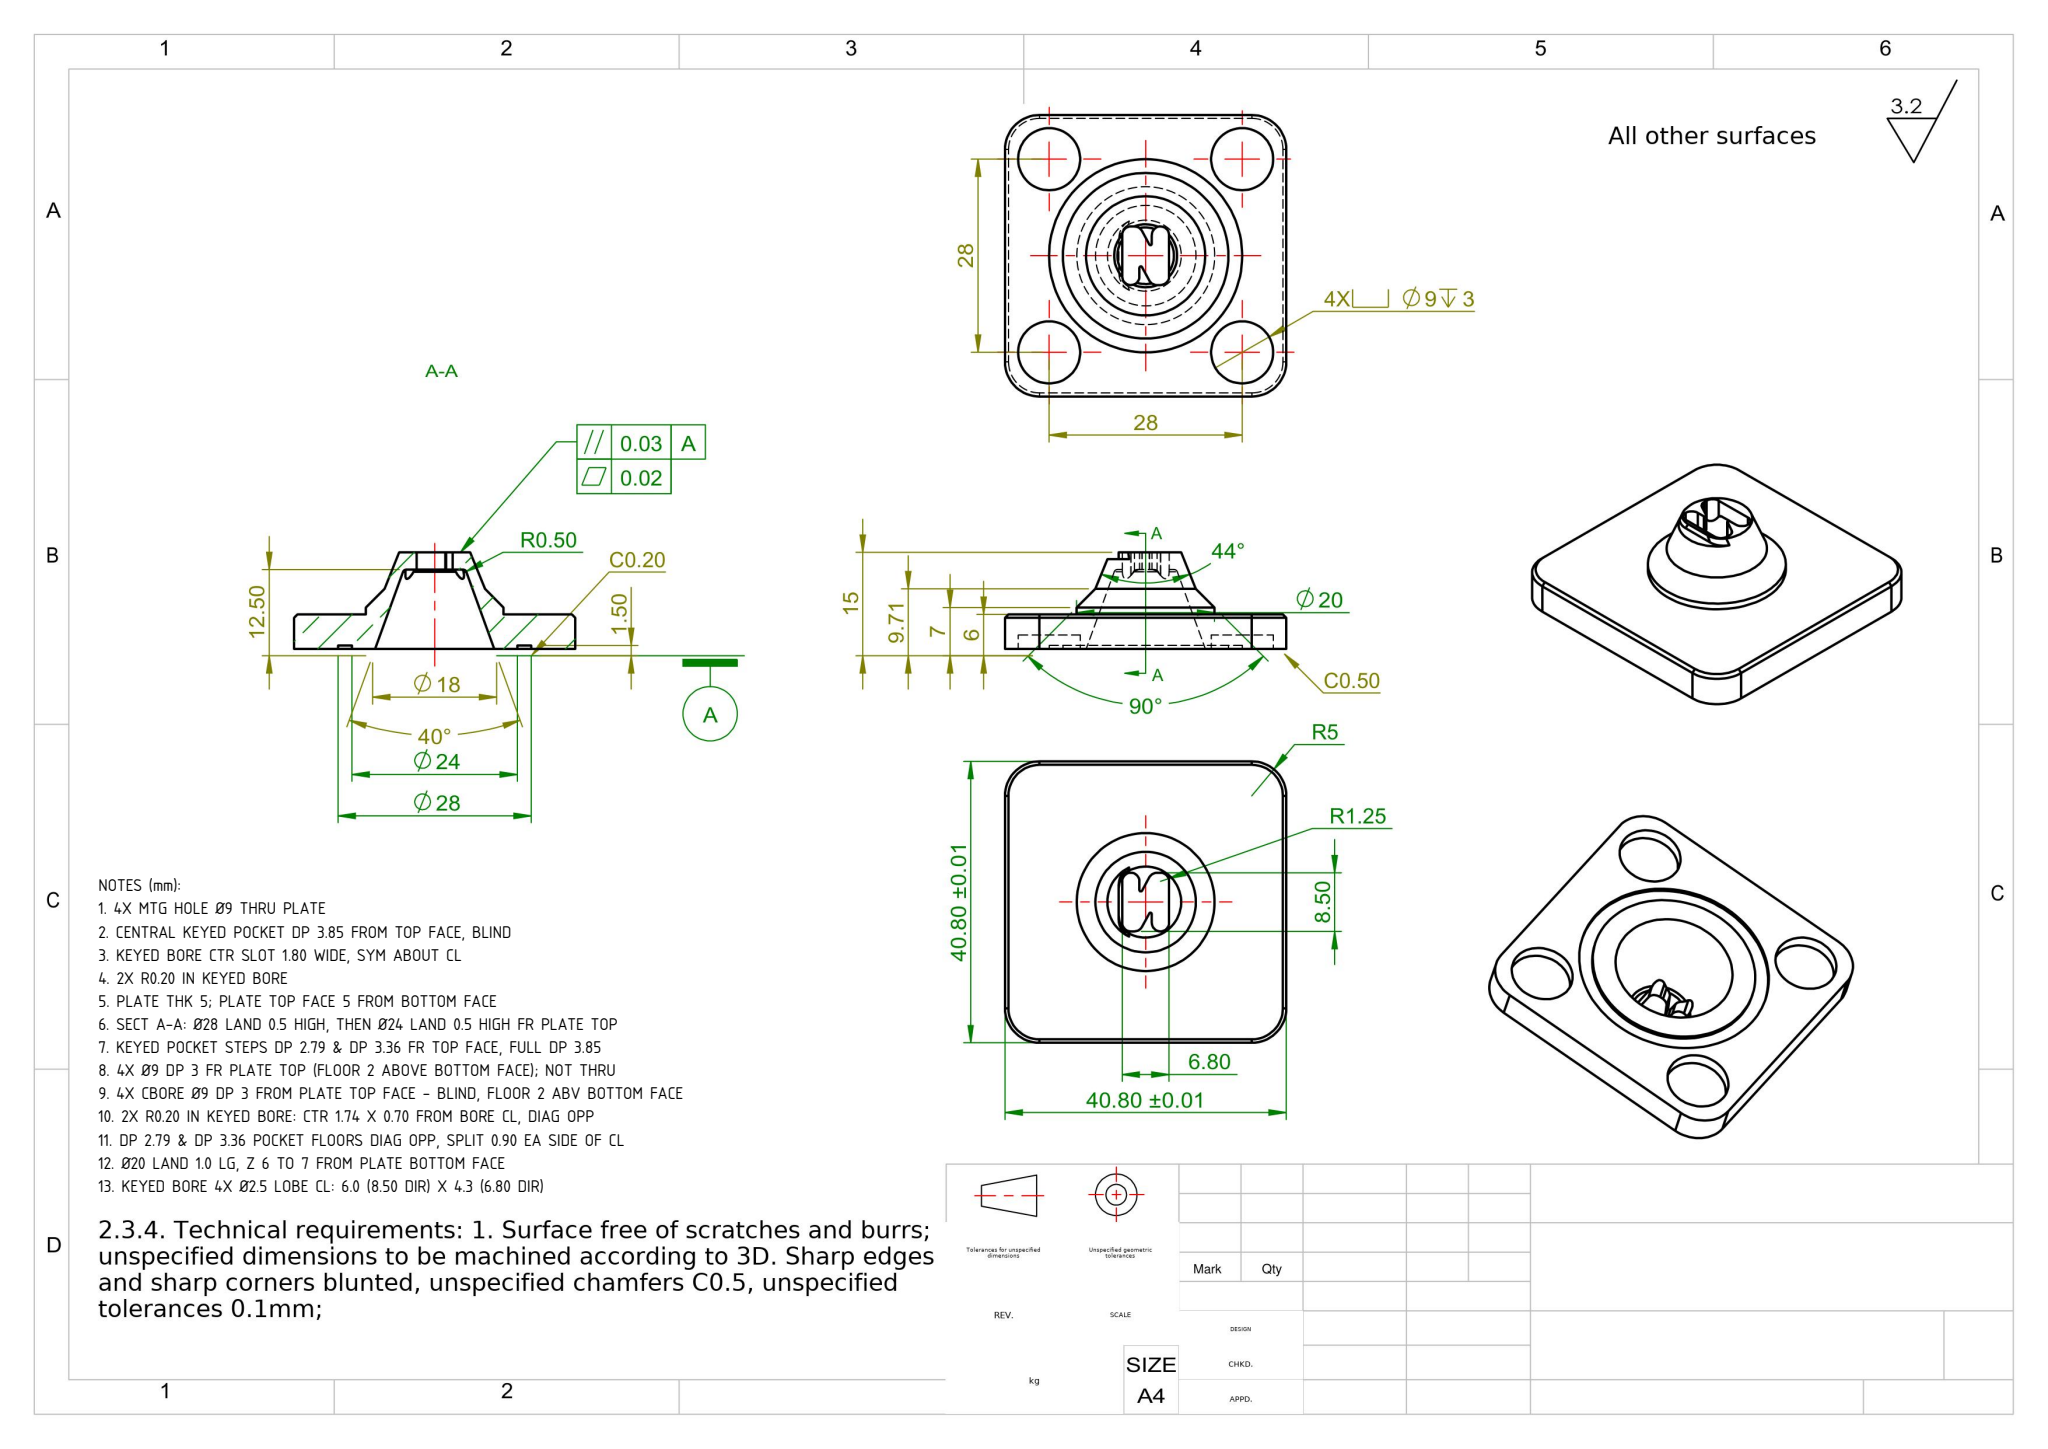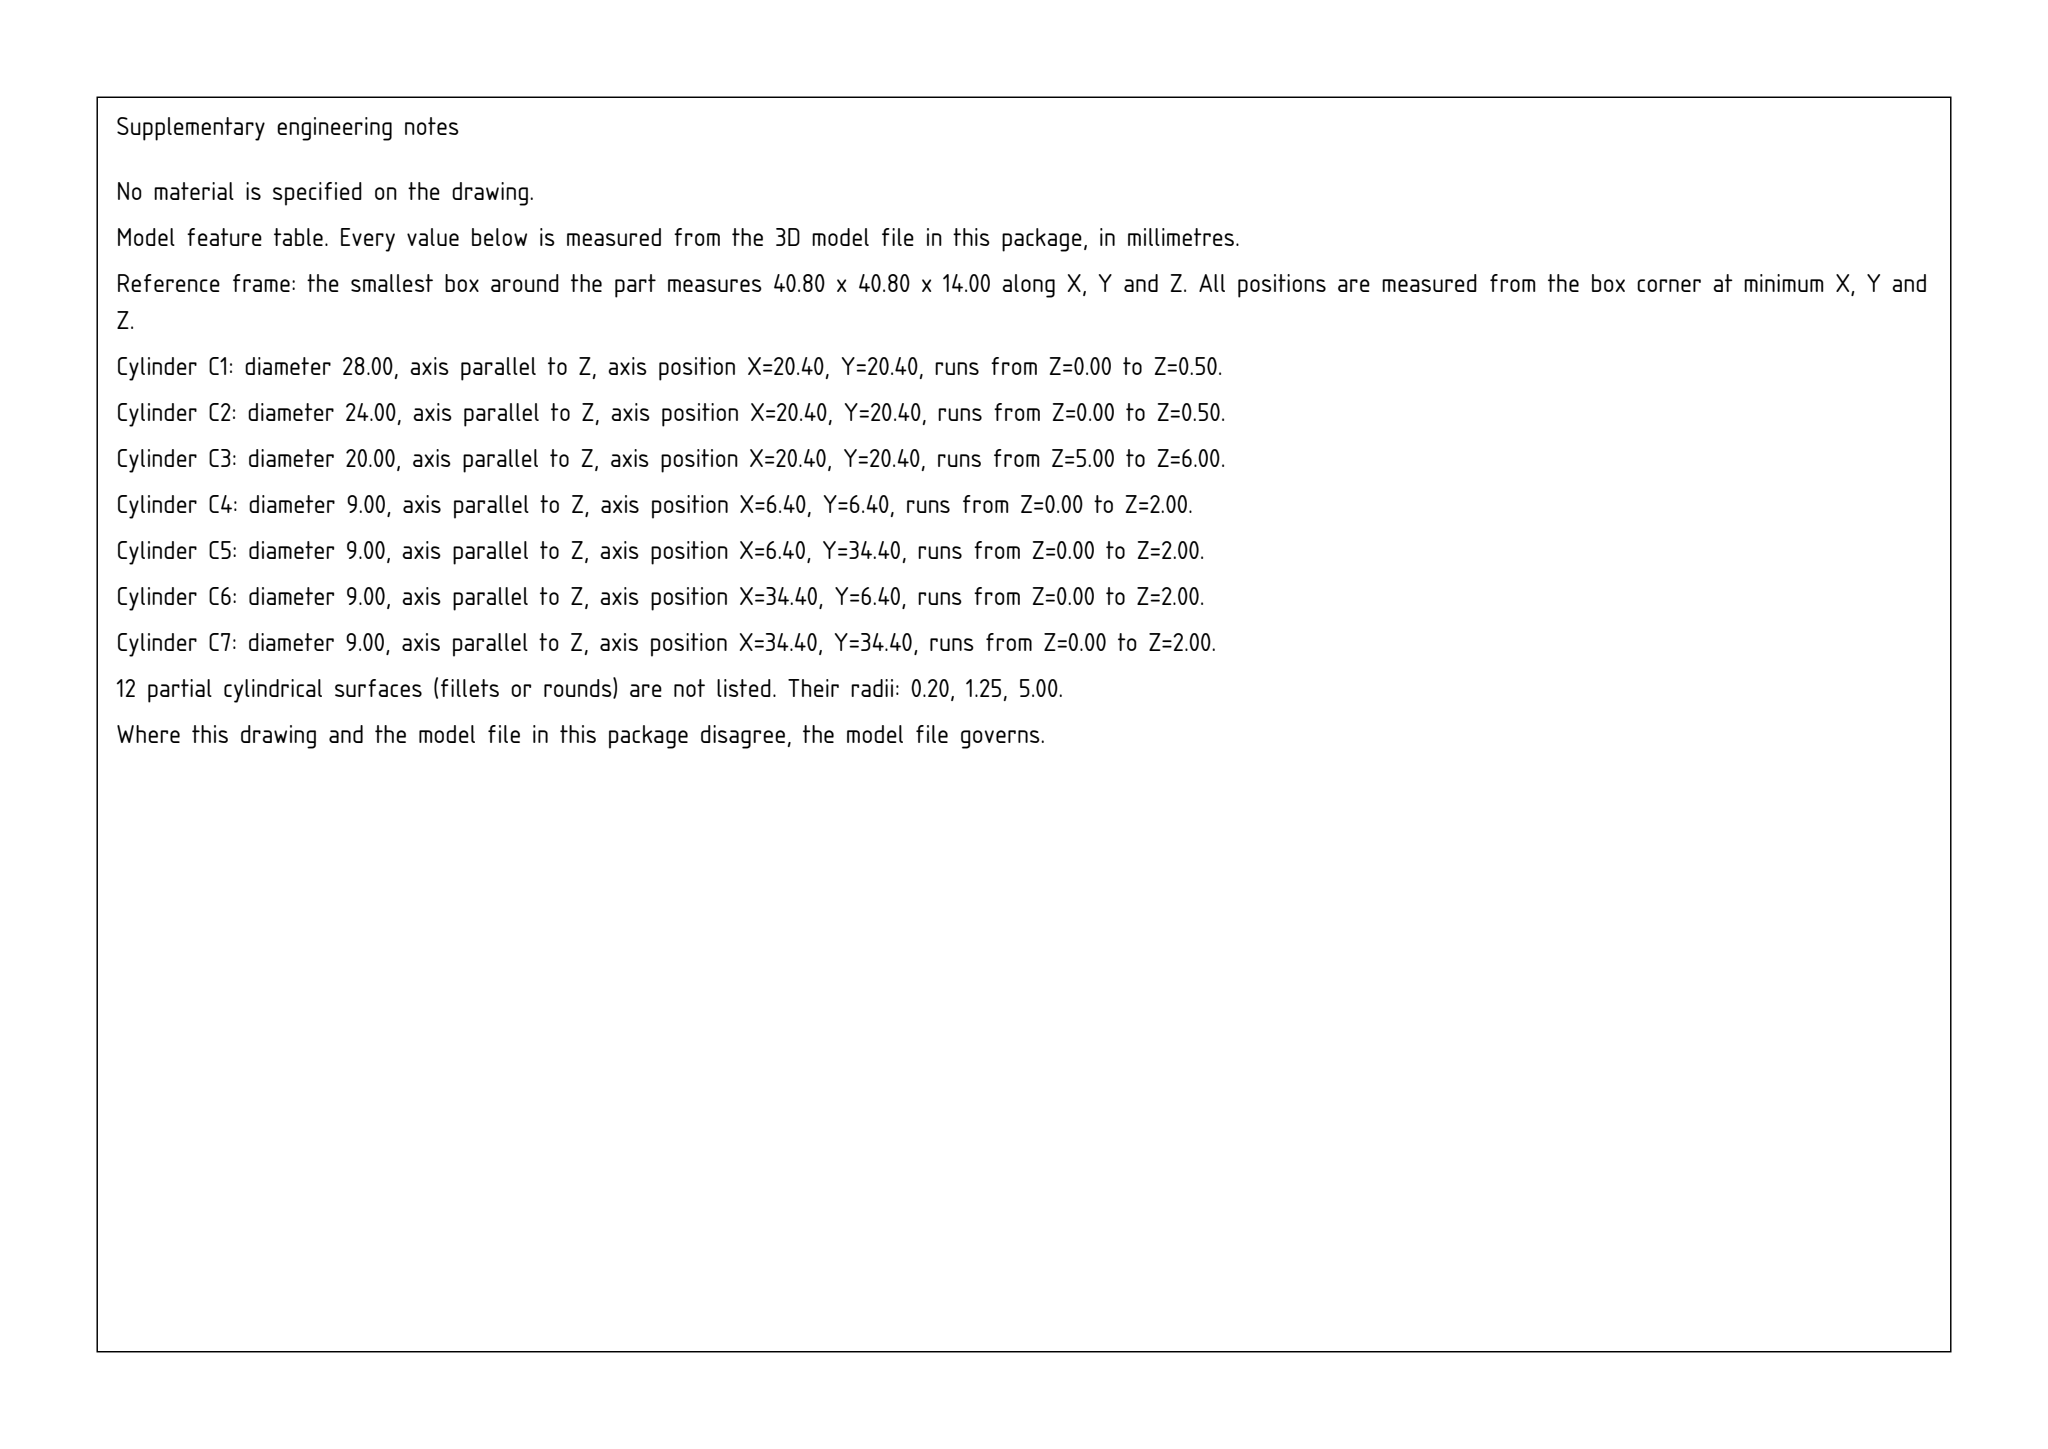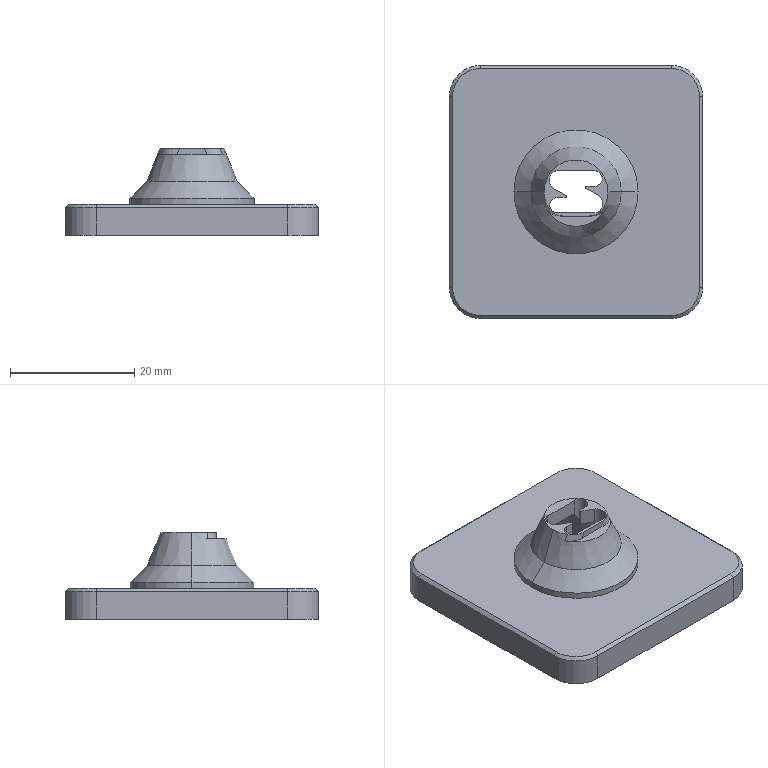Part | SolidWorks | mm | 1 solid | 77 faces | box 40.8 x 40.8 x 14 mm | volume 7477 mm3 | plane 31 | cylinder 29 | cone 10 | torus 5 | spline 2 | commonest cylinder face diameters 9 x8 2.5 x8 10 x4 0.4 x3 24 x2 28 x2 20 x2
Drawing notes:
4X MTG HOLE Ø9 THRU PLATE | from the solid: Ø9.0 z-cyls at (6.4,6.4),(6.4,34.4),(34.4,6.4),(34.4,34.4), 2 faces L2.0 each = full plate thk; 90° chamfers ref Ø9 both ends; no blind bottom face
CENTRAL KEYED POCKET DP 3.85 FROM TOP FACE, BLIND | from the solid: max Ø2.5 lobe length 3.85 from top z=14.949 (15 level) to z=11.10; no lobe breaks into Ø20 underside bore
KEYED BORE CTR SLOT 1.80 WIDE, SYM ABOUT CL | from the solid: axis planes y=19.5 and y=21.3, both 0.9 from part CL y=20.4
2X R0.20 IN KEYED BORE | from the solid: Ø0.4 z-cyls at (18.66,19.7) and (22.14,21.1), L2.5
PLATE THK 5; PLATE TOP FACE 5 FROM BOTTOM FACE | from the solid: z-plane at 5.0 is plate top; bbox z 0-14.949, base face z=0
SECT A-A: Ø28 LAND 0.5 HIGH, THEN Ø24 LAND 0.5 HIGH FR PLATE TOP | from the solid: cyl Ø28 len 0.5 and Ø24 len 0.5 above z=5; Ø20 len 1.0 to z=7
KEYED POCKET STEPS DP 2.79 & DP 3.36 FR TOP FACE, FULL DP 3.85 | from the solid: Ø2.5 z-cyls of length 2.79, 3.36 and 3.85 at pocket corners
4X Ø9 DP 3 FR PLATE TOP (FLOOR 2 ABOVE BOTTOM FACE); NOT THRU | from the solid: Ø9 z-cyls at 28 sq pattern, floor z-plane 2.0 x4, plate top z=5
4X CBORE Ø9 DP 3 FROM PLATE TOP FACE - BLIND, FLOOR 2 ABV BOTTOM FACE | from the solid: Ø9 holes at (6.4/34.4, 6.4/34.4), cyl len 2.0 + 90° point, floor plane z=2.0; plate top face z=5.0, bottom face z=0 (plate 5 thk) -> depth 3, not thru
2X R0.20 IN KEYED BORE: CTR 1.74 X 0.70 FROM BORE CL, DIAG OPP | from the solid: R0.2 (Ø0.4) cyls, axis z, at (18.66,19.70) and (22.14,21.10); bore CL (20.4,20.4) -> ±1.74, ±0.70, 180° apart
DP 2.79 & DP 3.36 POCKET FLOORS DIAG OPP, SPLIT 0.90 EA SIDE OF CL | from the solid: step walls at y=19.5 and 21.3 (=CL 20.4 ±0.90); 2.79 deep lobes at (17.4,22.04)&(23.4,18.76), 3.36 deep at (17.4,18.25)&(23.4,22.55)
Ø20 LAND 1.0 LG, Z 6 TO 7 FROM PLATE BOTTOM FACE | from the solid: Ø20 cyl, axis z at (20.4,20.4), length 1.0; between lower 90° cone and upper 90°/44° cones giving top Ø10.3 at z=14.95
KEYED BORE 4X Ø2.5 LOBE CL: 6.0 (8.50 DIR) X 4.3 (6.80 DIR) | from the solid: Ø2.5 lobe axes at x=17.4 & 23.4 (6.0 apart, env 8.5), y=18.25 & 22.55 (4.3 apart, env 6.8), centred on (20.4,20.4)